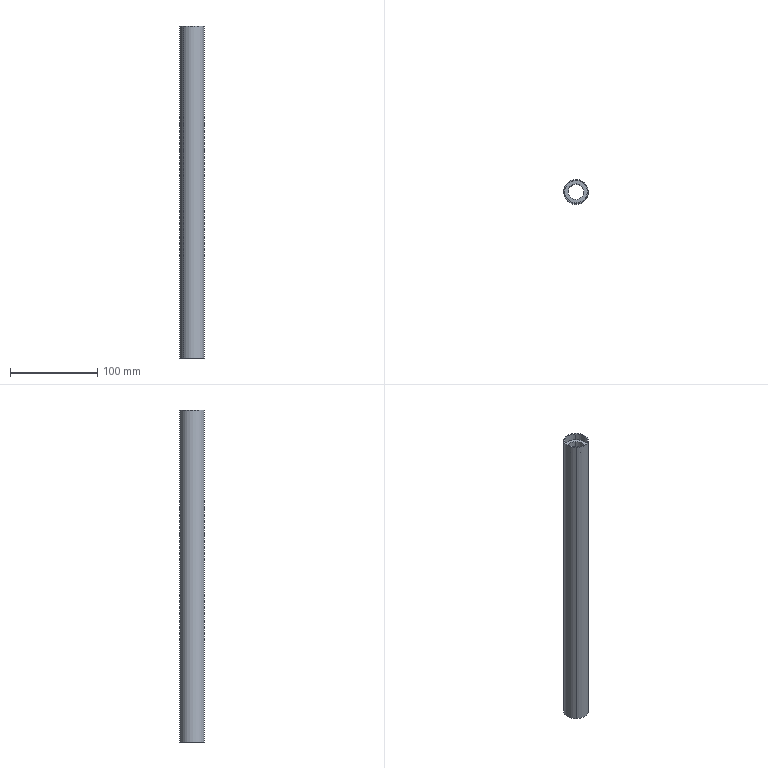Component | SolidWorks | Roller1-1-2 | 1 solid | 12 faces | box 28 x 28 x 380 mm | volume 132864 mm3 | cylinder 8 | plane 4 | commonest cylinder face diameters 26 x4 18 x2 28 x2
build123d program:
from build123d import *

# Parameters (mm, degrees)
MOVE_FACE1_BY = 1


with BuildPart() as part:
    # Sketch1 → Revolve1 (revolve)
    with BuildSketch(Plane(origin=(0, 0, 0), x_dir=(-1, 0, 0), z_dir=(0, 0, -1)), mode=Mode.PRIVATE) as revolve1_sk:
        Polygon((-182, 13), (-182, 9), (182, 9), (182, 13), (190, 13), (190, 15), (-190, 15), (-190, 13), align=None)
    revolve(revolve1_sk.sketch.rotate(Axis((190, 0, 0), (-1, 0, 0)), 270), axis=Axis((190, 0, 0), (-1, 0, 0)))

    # Move Face1: a curved face moved inward by 1.0
    add(Solid.thicken(part.faces().sort_by_distance((0, 0, -15))[0], -MOVE_FACE1_BY), mode=Mode.SUBTRACT)


solid = part.part

# Placed as in the assembly
solid = solid.moved(Location((-180.767, 560.9, 0), (0, 90, 0)))
STEP:
#1=COLOUR_RGB('',0.7922,0.8196,0.9333);
#2=FILL_AREA_STYLE_COLOUR('',#1);
#3=FILL_AREA_STYLE('',(#2));
#4=SURFACE_STYLE_FILL_AREA(#3);
#5=SURFACE_SIDE_STYLE('',(#4));
#6=SURFACE_STYLE_USAGE(.BOTH.,#5);
#7=PRESENTATION_STYLE_ASSIGNMENT((#6));
#8=CARTESIAN_POINT('',(-7.363,21.828,-7.165));
#9=VERTEX_POINT('',#8);
#10=CARTESIAN_POINT('',(-6.871,22.338,-7.165));
#11=VERTEX_POINT('',#10);
#12=CARTESIAN_POINT('',(-7.117,22.083,-7.165));
#13=DIRECTION('',(-0.,0.,1.));
#14=DIRECTION('',(0.694,0.72,0.));
#15=AXIS2_PLACEMENT_3D('',#12,#13,#14);
#16=CIRCLE('',#15,0.3543);
#17=EDGE_CURVE('',#9,#11,#16,.T.);
#18=ORIENTED_EDGE('',*,*,#17,.F.);
#19=CARTESIAN_POINT('',(-7.363,21.828,7.165));
#20=VERTEX_POINT('',#19);
#21=CARTESIAN_POINT('',(-7.363,21.828,-7.48));
#22=DIRECTION('',(-0.,0.,1.));
#23=VECTOR('',#22,39.37);
#24=LINE('',#21,#23);
#25=EDGE_CURVE('',#9,#20,#24,.T.);
#26=ORIENTED_EDGE('',*,*,#25,.T.);
#27=CARTESIAN_POINT('',(-6.871,22.338,7.165));
#28=VERTEX_POINT('',#27);
#29=CARTESIAN_POINT('',(-7.117,22.083,7.165));
#30=DIRECTION('',(-0.,0.,1.));
#31=DIRECTION('',(0.694,0.72,0.));
#32=AXIS2_PLACEMENT_3D('',#29,#30,#31);
#33=CIRCLE('',#32,0.3543);
#34=EDGE_CURVE('',#20,#28,#33,.T.);
#35=ORIENTED_EDGE('',*,*,#34,.T.);
#36=CARTESIAN_POINT('',(-6.871,22.338,-7.48));
#37=DIRECTION('',(-0.,0.,1.));
#38=VECTOR('',#37,39.37);
#39=LINE('',#36,#38);
#40=EDGE_CURVE('',#11,#28,#39,.T.);
#41=ORIENTED_EDGE('',*,*,#40,.F.);
#42=EDGE_LOOP('',(#18,#26,#35,#41));
#43=FACE_OUTER_BOUND('',#42,.T.);
#44=CARTESIAN_POINT('',(-7.117,22.083,-7.48));
#45=DIRECTION('',(-0.,0.,1.));
#46=DIRECTION('',(0.694,0.72,0.));
#47=AXIS2_PLACEMENT_3D('',#44,#45,#46);
#48=CYLINDRICAL_SURFACE('',#47,0.3543);
#49=ADVANCED_FACE('',(#43),#48,.F.);
#50=CARTESIAN_POINT('',(-7.472,21.714,7.165));
#51=VERTEX_POINT('',#50);
#52=CARTESIAN_POINT('',(-6.762,22.451,7.165));
#53=VERTEX_POINT('',#52);
#54=CARTESIAN_POINT('',(-7.117,22.083,7.165));
#55=DIRECTION('',(-0.,0.,1.));
#56=DIRECTION('',(0.694,0.72,0.));
#57=AXIS2_PLACEMENT_3D('',#54,#55,#56);
#58=CIRCLE('',#57,0.5118);
#59=EDGE_CURVE('',#51,#53,#58,.T.);
#60=ORIENTED_EDGE('',*,*,#59,.F.);
#61=CARTESIAN_POINT('',(-7.472,21.714,7.48));
#62=VERTEX_POINT('',#61);
#63=CARTESIAN_POINT('',(-7.472,21.714,-7.48));
#64=DIRECTION('',(-0.,0.,1.));
#65=VECTOR('',#64,39.37);
#66=LINE('',#63,#65);
#67=EDGE_CURVE('',#51,#62,#66,.T.);
#68=ORIENTED_EDGE('',*,*,#67,.T.);
#69=CARTESIAN_POINT('',(-6.762,22.451,7.48));
#70=VERTEX_POINT('',#69);
#71=CARTESIAN_POINT('',(-7.117,22.083,7.48));
#72=DIRECTION('',(-0.,0.,1.));
#73=DIRECTION('',(0.694,0.72,0.));
#74=AXIS2_PLACEMENT_3D('',#71,#72,#73);
#75=CIRCLE('',#74,0.5118);
#76=EDGE_CURVE('',#62,#70,#75,.T.);
#77=ORIENTED_EDGE('',*,*,#76,.T.);
#78=CARTESIAN_POINT('',(-6.762,22.451,-7.48));
#79=DIRECTION('',(-0.,0.,1.));
#80=VECTOR('',#79,39.37);
#81=LINE('',#78,#80);
#82=EDGE_CURVE('',#53,#70,#81,.T.);
#83=ORIENTED_EDGE('',*,*,#82,.F.);
#84=EDGE_LOOP('',(#60,#68,#77,#83));
#85=FACE_OUTER_BOUND('',#84,.T.);
#86=CARTESIAN_POINT('',(-7.117,22.083,-7.48));
#87=DIRECTION('',(-0.,0.,1.));
#88=DIRECTION('',(0.694,0.72,0.));
#89=AXIS2_PLACEMENT_3D('',#86,#87,#88);
#90=CYLINDRICAL_SURFACE('',#89,0.5118);
#91=ADVANCED_FACE('',(#85),#90,.F.);
#92=CARTESIAN_POINT('',(-6.734,22.48,-7.48));
#93=VERTEX_POINT('',#92);
#94=CARTESIAN_POINT('',(-7.499,21.686,-7.48));
#95=VERTEX_POINT('',#94);
#96=CARTESIAN_POINT('',(-7.117,22.083,-7.48));
#97=DIRECTION('',(-0.,0.,1.));
#98=DIRECTION('',(-0.694,-0.72,0.));
#99=AXIS2_PLACEMENT_3D('',#96,#97,#98);
#100=CIRCLE('',#99,0.5512);
#101=EDGE_CURVE('',#93,#95,#100,.T.);
#102=ORIENTED_EDGE('',*,*,#101,.T.);
#103=CARTESIAN_POINT('',(-7.499,21.686,7.48));
#104=VERTEX_POINT('',#103);
#105=CARTESIAN_POINT('',(-7.499,21.686,-7.48));
#106=DIRECTION('',(-0.,0.,1.));
#107=VECTOR('',#106,39.37);
#108=LINE('',#105,#107);
#109=EDGE_CURVE('',#95,#104,#108,.T.);
#110=ORIENTED_EDGE('',*,*,#109,.T.);
#111=CARTESIAN_POINT('',(-6.734,22.48,7.48));
#112=VERTEX_POINT('',#111);
#113=CARTESIAN_POINT('',(-7.117,22.083,7.48));
#114=DIRECTION('',(-0.,0.,1.));
#115=DIRECTION('',(0.694,0.72,0.));
#116=AXIS2_PLACEMENT_3D('',#113,#114,#115);
#117=CIRCLE('',#116,0.5512);
#118=EDGE_CURVE('',#112,#104,#117,.T.);
#119=ORIENTED_EDGE('',*,*,#118,.F.);
#120=CARTESIAN_POINT('',(-6.734,22.48,-7.48));
#121=DIRECTION('',(-0.,0.,1.));
#122=VECTOR('',#121,39.37);
#123=LINE('',#120,#122);
#124=EDGE_CURVE('',#93,#112,#123,.T.);
#125=ORIENTED_EDGE('',*,*,#124,.F.);
#126=EDGE_LOOP('',(#102,#110,#119,#125));
#127=FACE_OUTER_BOUND('',#126,.T.);
#128=CARTESIAN_POINT('',(-7.117,22.083,-7.48));
#129=DIRECTION('',(-0.,0.,1.));
#130=DIRECTION('',(0.694,0.72,0.));
#131=AXIS2_PLACEMENT_3D('',#128,#129,#130);
#132=CYLINDRICAL_SURFACE('',#131,0.5512);
#133=ADVANCED_FACE('',(#127),#132,.T.);
#134=CARTESIAN_POINT('',(-7.472,21.714,-7.48));
#135=VERTEX_POINT('',#134);
#136=CARTESIAN_POINT('',(-6.762,22.451,-7.48));
#137=VERTEX_POINT('',#136);
#138=CARTESIAN_POINT('',(-7.117,22.083,-7.48));
#139=DIRECTION('',(-0.,0.,1.));
#140=DIRECTION('',(0.694,0.72,0.));
#141=AXIS2_PLACEMENT_3D('',#138,#139,#140);
#142=CIRCLE('',#141,0.5118);
#143=EDGE_CURVE('',#135,#137,#142,.T.);
#144=ORIENTED_EDGE('',*,*,#143,.F.);
#145=CARTESIAN_POINT('',(-7.472,21.714,-7.165));
#146=VERTEX_POINT('',#145);
#147=CARTESIAN_POINT('',(-7.472,21.714,-7.48));
#148=DIRECTION('',(-0.,0.,1.));
#149=VECTOR('',#148,39.37);
#150=LINE('',#147,#149);
#151=EDGE_CURVE('',#135,#146,#150,.T.);
#152=ORIENTED_EDGE('',*,*,#151,.T.);
#153=CARTESIAN_POINT('',(-6.762,22.451,-7.165));
#154=VERTEX_POINT('',#153);
#155=CARTESIAN_POINT('',(-7.117,22.083,-7.165));
#156=DIRECTION('',(-0.,0.,1.));
#157=DIRECTION('',(0.694,0.72,0.));
#158=AXIS2_PLACEMENT_3D('',#155,#156,#157);
#159=CIRCLE('',#158,0.5118);
#160=EDGE_CURVE('',#146,#154,#159,.T.);
#161=ORIENTED_EDGE('',*,*,#160,.T.);
#162=CARTESIAN_POINT('',(-6.762,22.451,-7.48));
#163=DIRECTION('',(-0.,0.,1.));
#164=VECTOR('',#163,39.37);
#165=LINE('',#162,#164);
#166=EDGE_CURVE('',#137,#154,#165,.T.);
#167=ORIENTED_EDGE('',*,*,#166,.F.);
#168=EDGE_LOOP('',(#144,#152,#161,#167));
#169=FACE_OUTER_BOUND('',#168,.T.);
#170=CARTESIAN_POINT('',(-7.117,22.083,-7.48));
#171=DIRECTION('',(-0.,0.,1.));
#172=DIRECTION('',(0.694,0.72,0.));
#173=AXIS2_PLACEMENT_3D('',#170,#171,#172);
#174=CYLINDRICAL_SURFACE('',#173,0.5118);
#175=ADVANCED_FACE('',(#169),#174,.F.);
#176=ORIENTED_EDGE('',*,*,#151,.F.);
#177=CARTESIAN_POINT('',(-7.117,22.083,-7.48));
#178=DIRECTION('',(-0.,0.,1.));
#179=DIRECTION('',(0.694,0.72,0.));
#180=AXIS2_PLACEMENT_3D('',#177,#178,#179);
#181=CIRCLE('',#180,0.5118);
#182=EDGE_CURVE('',#137,#135,#181,.T.);
#183=ORIENTED_EDGE('',*,*,#182,.F.);
#184=ORIENTED_EDGE('',*,*,#166,.T.);
#185=CARTESIAN_POINT('',(-7.117,22.083,-7.165));
#186=DIRECTION('',(-0.,0.,1.));
#187=DIRECTION('',(0.694,0.72,0.));
#188=AXIS2_PLACEMENT_3D('',#185,#186,#187);
#189=CIRCLE('',#188,0.5118);
#190=EDGE_CURVE('',#154,#146,#189,.T.);
#191=ORIENTED_EDGE('',*,*,#190,.T.);
#192=EDGE_LOOP('',(#176,#183,#184,#191));
#193=FACE_OUTER_BOUND('',#192,.T.);
#194=CARTESIAN_POINT('',(-7.117,22.083,-7.48));
#195=DIRECTION('',(-0.,0.,1.));
#196=DIRECTION('',(0.694,0.72,0.));
#197=AXIS2_PLACEMENT_3D('',#194,#195,#196);
#198=CYLINDRICAL_SURFACE('',#197,0.5118);
#199=ADVANCED_FACE('',(#193),#198,.F.);
#200=ORIENTED_EDGE('',*,*,#182,.T.);
#201=ORIENTED_EDGE('',*,*,#143,.T.);
#202=EDGE_LOOP('',(#200,#201));
#203=FACE_BOUND('',#202,.T.);
#204=ORIENTED_EDGE('',*,*,#101,.F.);
#205=CARTESIAN_POINT('',(-7.117,22.083,-7.48));
#206=DIRECTION('',(-0.,0.,1.));
#207=DIRECTION('',(-0.694,-0.72,0.));
#208=AXIS2_PLACEMENT_3D('',#205,#206,#207);
#209=CIRCLE('',#208,0.5512);
#210=EDGE_CURVE('',#95,#93,#209,.T.);
#211=ORIENTED_EDGE('',*,*,#210,.F.);
#212=EDGE_LOOP('',(#204,#211));
#213=FACE_OUTER_BOUND('',#212,.T.);
#214=CARTESIAN_POINT('',(-7.542,22.493,-7.48));
#215=DIRECTION('',(0.,-0.,-1.));
#216=DIRECTION('',(-0.694,-0.72,0.));
#217=AXIS2_PLACEMENT_3D('',#214,#215,#216);
#218=PLANE('',#217);
#219=ADVANCED_FACE('',(#203,#213),#218,.T.);
#220=ORIENTED_EDGE('',*,*,#109,.F.);
#221=ORIENTED_EDGE('',*,*,#210,.T.);
#222=ORIENTED_EDGE('',*,*,#124,.T.);
#223=CARTESIAN_POINT('',(-7.117,22.083,7.48));
#224=DIRECTION('',(-0.,0.,1.));
#225=DIRECTION('',(0.694,0.72,0.));
#226=AXIS2_PLACEMENT_3D('',#223,#224,#225);
#227=CIRCLE('',#226,0.5512);
#228=EDGE_CURVE('',#104,#112,#227,.T.);
#229=ORIENTED_EDGE('',*,*,#228,.F.);
#230=EDGE_LOOP('',(#220,#221,#222,#229));
#231=FACE_OUTER_BOUND('',#230,.T.);
#232=CARTESIAN_POINT('',(-7.117,22.083,-7.48));
#233=DIRECTION('',(-0.,0.,1.));
#234=DIRECTION('',(0.694,0.72,0.));
#235=AXIS2_PLACEMENT_3D('',#232,#233,#234);
#236=CYLINDRICAL_SURFACE('',#235,0.5512);
#237=ADVANCED_FACE('',(#231),#236,.T.);
#238=ORIENTED_EDGE('',*,*,#118,.T.);
#239=ORIENTED_EDGE('',*,*,#228,.T.);
#240=EDGE_LOOP('',(#238,#239));
#241=FACE_OUTER_BOUND('',#240,.T.);
#242=CARTESIAN_POINT('',(-7.117,22.083,7.48));
#243=DIRECTION('',(-0.,0.,1.));
#244=DIRECTION('',(0.694,0.72,0.));
#245=AXIS2_PLACEMENT_3D('',#242,#243,#244);
#246=CIRCLE('',#245,0.5118);
#247=EDGE_CURVE('',#70,#62,#246,.T.);
#248=ORIENTED_EDGE('',*,*,#247,.F.);
#249=ORIENTED_EDGE('',*,*,#76,.F.);
#250=EDGE_LOOP('',(#248,#249));
#251=FACE_BOUND('',#250,.T.);
#252=CARTESIAN_POINT('',(-7.485,22.438,7.48));
#253=DIRECTION('',(-0.,0.,1.));
#254=DIRECTION('',(0.694,0.72,0.));
#255=AXIS2_PLACEMENT_3D('',#252,#253,#254);
#256=PLANE('',#255);
#257=ADVANCED_FACE('',(#241,#251),#256,.T.);
#258=ORIENTED_EDGE('',*,*,#67,.F.);
#259=CARTESIAN_POINT('',(-7.117,22.083,7.165));
#260=DIRECTION('',(-0.,0.,1.));
#261=DIRECTION('',(0.694,0.72,0.));
#262=AXIS2_PLACEMENT_3D('',#259,#260,#261);
#263=CIRCLE('',#262,0.5118);
#264=EDGE_CURVE('',#53,#51,#263,.T.);
#265=ORIENTED_EDGE('',*,*,#264,.F.);
#266=ORIENTED_EDGE('',*,*,#82,.T.);
#267=ORIENTED_EDGE('',*,*,#247,.T.);
#268=EDGE_LOOP('',(#258,#265,#266,#267));
#269=FACE_OUTER_BOUND('',#268,.T.);
#270=CARTESIAN_POINT('',(-7.117,22.083,-7.48));
#271=DIRECTION('',(-0.,0.,1.));
#272=DIRECTION('',(0.694,0.72,0.));
#273=AXIS2_PLACEMENT_3D('',#270,#271,#272);
#274=CYLINDRICAL_SURFACE('',#273,0.5118);
#275=ADVANCED_FACE('',(#269),#274,.F.);
#276=ORIENTED_EDGE('',*,*,#264,.T.);
#277=ORIENTED_EDGE('',*,*,#59,.T.);
#278=EDGE_LOOP('',(#276,#277));
#279=FACE_OUTER_BOUND('',#278,.T.);
#280=CARTESIAN_POINT('',(-7.117,22.083,7.165));
#281=DIRECTION('',(-0.,0.,1.));
#282=DIRECTION('',(0.694,0.72,0.));
#283=AXIS2_PLACEMENT_3D('',#280,#281,#282);
#284=CIRCLE('',#283,0.3543);
#285=EDGE_CURVE('',#28,#20,#284,.T.);
#286=ORIENTED_EDGE('',*,*,#285,.F.);
#287=ORIENTED_EDGE('',*,*,#34,.F.);
#288=EDGE_LOOP('',(#286,#287));
#289=FACE_BOUND('',#288,.T.);
#290=CARTESIAN_POINT('',(-7.372,22.329,7.165));
#291=DIRECTION('',(-0.,0.,1.));
#292=DIRECTION('',(0.694,0.72,0.));
#293=AXIS2_PLACEMENT_3D('',#290,#291,#292);
#294=PLANE('',#293);
#295=ADVANCED_FACE('',(#279,#289),#294,.T.);
#296=ORIENTED_EDGE('',*,*,#25,.F.);
#297=CARTESIAN_POINT('',(-7.117,22.083,-7.165));
#298=DIRECTION('',(-0.,0.,1.));
#299=DIRECTION('',(0.694,0.72,0.));
#300=AXIS2_PLACEMENT_3D('',#297,#298,#299);
#301=CIRCLE('',#300,0.3543);
#302=EDGE_CURVE('',#11,#9,#301,.T.);
#303=ORIENTED_EDGE('',*,*,#302,.F.);
#304=ORIENTED_EDGE('',*,*,#40,.T.);
#305=ORIENTED_EDGE('',*,*,#285,.T.);
#306=EDGE_LOOP('',(#296,#303,#304,#305));
#307=FACE_OUTER_BOUND('',#306,.T.);
#308=CARTESIAN_POINT('',(-7.117,22.083,-7.48));
#309=DIRECTION('',(-0.,0.,1.));
#310=DIRECTION('',(0.694,0.72,0.));
#311=AXIS2_PLACEMENT_3D('',#308,#309,#310);
#312=CYLINDRICAL_SURFACE('',#311,0.3543);
#313=ADVANCED_FACE('',(#307),#312,.F.);
#314=ORIENTED_EDGE('',*,*,#302,.T.);
#315=ORIENTED_EDGE('',*,*,#17,.T.);
#316=EDGE_LOOP('',(#314,#315));
#317=FACE_BOUND('',#316,.T.);
#318=ORIENTED_EDGE('',*,*,#190,.F.);
#319=ORIENTED_EDGE('',*,*,#160,.F.);
#320=EDGE_LOOP('',(#318,#319));
#321=FACE_OUTER_BOUND('',#320,.T.);
#322=CARTESIAN_POINT('',(-7.485,22.438,-7.165));
#323=DIRECTION('',(0.,-0.,-1.));
#324=DIRECTION('',(-0.694,-0.72,0.));
#325=AXIS2_PLACEMENT_3D('',#322,#323,#324);
#326=PLANE('',#325);
#327=ADVANCED_FACE('',(#317,#321),#326,.T.);
#328=CLOSED_SHELL('',(#49,#91,#133,#175,#199,#219,#237,#257,#275,#295,#313,#327));
#329=MANIFOLD_SOLID_BREP('',#328);
#330=STYLED_ITEM('',(#7),#329);
#331=(LENGTH_UNIT()NAMED_UNIT(*)SI_UNIT($,.METRE.));
#332=LENGTH_MEASURE_WITH_UNIT(LENGTH_MEASURE(0.0254),#331);
#333=DIMENSIONAL_EXPONENTS(1.,0.,0.,0.,0.,0.,0.);
#334=(CONVERSION_BASED_UNIT('',#332)LENGTH_UNIT()NAMED_UNIT(#333));
#335=UNCERTAINTY_MEASURE_WITH_UNIT(LENGTH_MEASURE(0.00001),#334,'','');
#336=(NAMED_UNIT(*)PLANE_ANGLE_UNIT()SI_UNIT($,.RADIAN.));
#337=(NAMED_UNIT(*)SI_UNIT($,.STERADIAN.)SOLID_ANGLE_UNIT());
#338=(GEOMETRIC_REPRESENTATION_CONTEXT(3)GLOBAL_UNCERTAINTY_ASSIGNED_CONTEXT((#335))GLOBAL_UNIT_ASSIGNED_CONTEXT((#334,#336,#337))REPRESENTATION_CONTEXT('',''));
#339=MECHANICAL_DESIGN_GEOMETRIC_PRESENTATION_REPRESENTATION('',(#330),#338);
#340=CARTESIAN_POINT('',(0.,0.,0.));
#341=DIRECTION('',(0.,0.,1.));
#342=DIRECTION('',(1.,0.,0.));
#343=AXIS2_PLACEMENT_3D('',#340,#341,#342);
#344=(LENGTH_UNIT()NAMED_UNIT(*)SI_UNIT($,.METRE.));
#345=LENGTH_MEASURE_WITH_UNIT(LENGTH_MEASURE(0.0254),#344);
#346=DIMENSIONAL_EXPONENTS(1.,0.,0.,0.,0.,0.,0.);
#347=(CONVERSION_BASED_UNIT('',#345)LENGTH_UNIT()NAMED_UNIT(#346));
#348=UNCERTAINTY_MEASURE_WITH_UNIT(LENGTH_MEASURE(0.00001),#347,'','');
#349=(NAMED_UNIT(*)PLANE_ANGLE_UNIT()SI_UNIT($,.RADIAN.));
#350=(NAMED_UNIT(*)SI_UNIT($,.STERADIAN.)SOLID_ANGLE_UNIT());
#351=(GEOMETRIC_REPRESENTATION_CONTEXT(3)GLOBAL_UNCERTAINTY_ASSIGNED_CONTEXT((#348))GLOBAL_UNIT_ASSIGNED_CONTEXT((#347,#349,#350))REPRESENTATION_CONTEXT('',''));
#352=ADVANCED_BREP_SHAPE_REPRESENTATION('',(#329,#343),#351);
#353=PRESENTATION_LAYER_ASSIGNMENT('','',(#330));